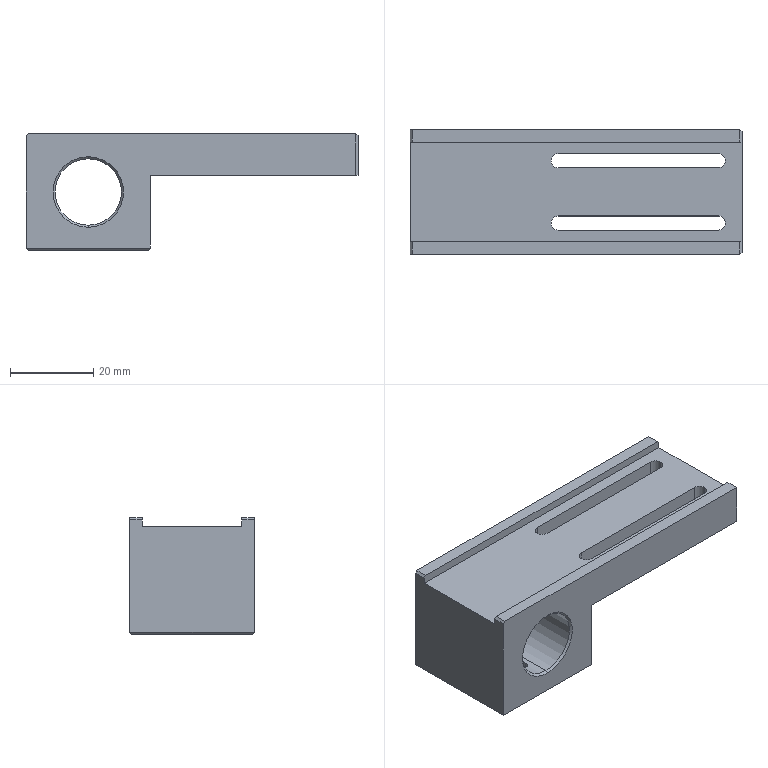Component | SolidWorks | JR-PL-JD-07Slider-1 | 1 solid | 64 faces | volume 27125 mm3 | plane 36 | cylinder 18 | cone 10 | commonest cylinder face diameters 6 x6 3.4 x6 3.3 x4 16 x2